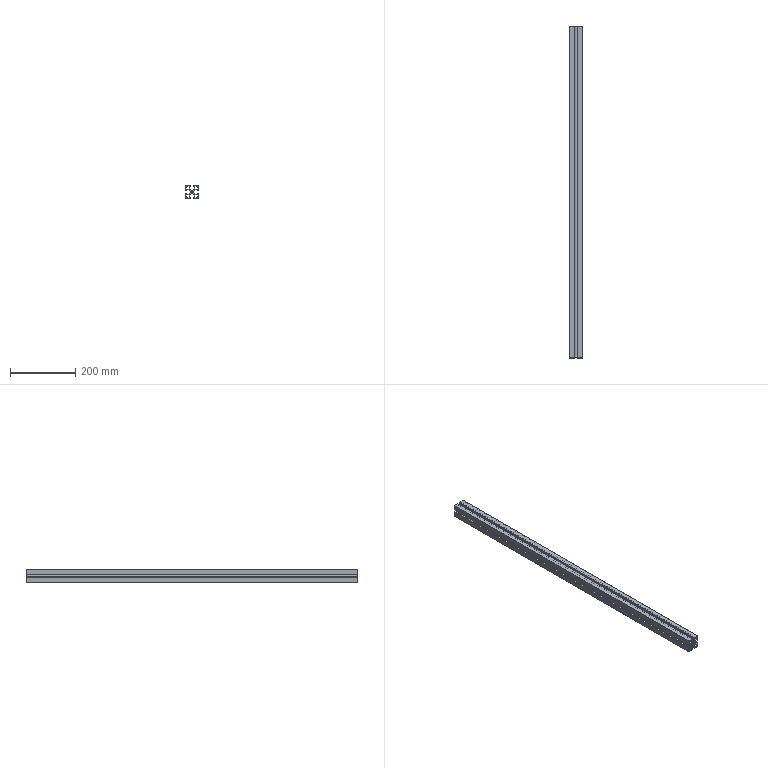Component | SolidWorks | AluminumProfile720-1 | 1 solid | 89 faces | box 40 x 1020 x 40 mm | volume 591676 mm3 | plane 82 | cylinder 7 | commonest cylinder face diameters 10.5 x5 6.8 x2 | material 6061 Alloy
build123d program:
from build123d import *

# Parameters (mm, degrees)
SKETCH1_W                  = 40
SKETCH1_H                  = 40
EXTRUDE1_DEPTH             = 1640
CUT_EXTRUDE1_DEPTH         = 1641.975
SKETCH3_R                  = 3.4
CUT_EXTRUDE2_DEPTH         = 1641.975
CIRPATTERN1_COUNT          = 4
EXTRUDE2_DEPTH             = 1641.975
CIRPATTERN2_COUNT          = 4
SKETCH5_W                  = 9
SKETCH5_H                  = 9
EXTRUDE3_DEPTH             = 1641.975
CIRPATTERN3_COUNT          = 4
M8X1_25_TAPPED_HOLE3_D     = 6.8
M8X1_25_TAPPED_HOLE3_DEPTH = 19.75
M8X1_25_TAPPED_HOLE3_TIP   = 2.043
SKETCH9_W                  = 177.591
SKETCH9_H                  = 2021.808
CUT_EXTRUDE3_DEPTH         = 1641.975


with BuildPart() as part:
    # Sketch1 → Extrude1 (new body)
    with BuildSketch(Plane.XY):
        with Locations((20, 20)):
            Rectangle(SKETCH1_W, SKETCH1_H)
    extrude(amount=EXTRUDE1_DEPTH)

    # Sketch2 → Cut-Extrude1 (cut, through all)
    with BuildSketch(Plane.XY.offset(1640)):
        Polygon((16, 40), (16, 36), (13, 36), (13, 29), (27, 29), (27, 36), (24, 36), (24, 40), align=None)
    cut_extrude1 = extrude(amount=-CUT_EXTRUDE1_DEPTH, mode=Mode.SUBTRACT)

    # Sketch3 → Cut-Extrude2 (cut, through all)
    with BuildSketch(Plane.XY.offset(1640)):
        with Locations((20, 20)):
            Circle(SKETCH3_R)
    extrude(amount=-CUT_EXTRUDE2_DEPTH, mode=Mode.SUBTRACT)

    # CirPattern1: Cut-Extrude1 ×4 about axis
    cirpattern1_axis = Axis((20, 20, 0), (0, 0, 1))
    for i in range(1, CIRPATTERN1_COUNT):
        add(cut_extrude1.rotate(cirpattern1_axis, i * 360 / CIRPATTERN1_COUNT), mode=Mode.SUBTRACT)

    # Sketch4 → Extrude2 (cut, through all)
    with BuildSketch(Plane.XY.offset(1640)):
        with BuildLine():
            Line((15.75, 29), (16.457, 28.293))
            Line((16.457, 28.293), (14.806, 26.641))
            Line((14.806, 26.641), (17.082, 24.365))
            ThreePointArc((17.082, 24.365), (20, 25.25), (22.918, 24.365))
            Line((22.918, 24.365), (25.194, 26.641))
            Line((25.194, 26.641), (23.543, 28.293))
            Line((23.543, 28.293), (24.25, 29))
            Line((24.25, 29), (15.75, 29))
        make_face()
    extrude2 = extrude(amount=-EXTRUDE2_DEPTH, mode=Mode.SUBTRACT)

    # CirPattern2: Extrude2 ×4 about axis
    cirpattern2_axis = Axis((20, 20, 0), (0, 0, 1))
    for i in range(1, CIRPATTERN2_COUNT):
        add(extrude2.rotate(cirpattern2_axis, i * 360 / CIRPATTERN2_COUNT), mode=Mode.SUBTRACT)

    # Sketch5 → Extrude3 (cut, through all)
    with BuildSketch(Plane.XY.offset(1640)):
        with Locations((6.5, 33.5)):
            Rectangle(SKETCH5_W, SKETCH5_H)
    extrude3 = extrude(amount=-EXTRUDE3_DEPTH, mode=Mode.SUBTRACT)

    # CirPattern3: Extrude3 ×4 about axis
    cirpattern3_axis = Axis((20, 20, 0), (0, 0, 1))
    for i in range(1, CIRPATTERN3_COUNT):
        add(extrude3.rotate(cirpattern3_axis, i * 360 / CIRPATTERN3_COUNT), mode=Mode.SUBTRACT)

    # M8x1.25 Tapped Hole3
    with Locations(Plane(origin=(20, 20, 1640), x_dir=(1, 0, 0), z_dir=(0, 0, 1))):
        with Locations((0, 0)):
            Hole(M8X1_25_TAPPED_HOLE3_D / 2, depth=M8X1_25_TAPPED_HOLE3_DEPTH)
            with Locations((0, 0, -(M8X1_25_TAPPED_HOLE3_DEPTH + M8X1_25_TAPPED_HOLE3_TIP / 2))):  # 118° drill point
                Cone(0, M8X1_25_TAPPED_HOLE3_D / 2, M8X1_25_TAPPED_HOLE3_TIP, mode=Mode.SUBTRACT)

    # Sketch9 → Cut-Extrude3 (cut, through all)
    with BuildSketch(Plane.XZ):
        with Locations((13.869, 2030.904)):
            Rectangle(SKETCH9_W, SKETCH9_H)
    extrude(amount=-CUT_EXTRUDE3_DEPTH, mode=Mode.SUBTRACT)


solid = part.part

# Placed as in the assembly
solid = solid.moved(Location((-768.352, 51.783, 643.715), (90, 0, 0)))